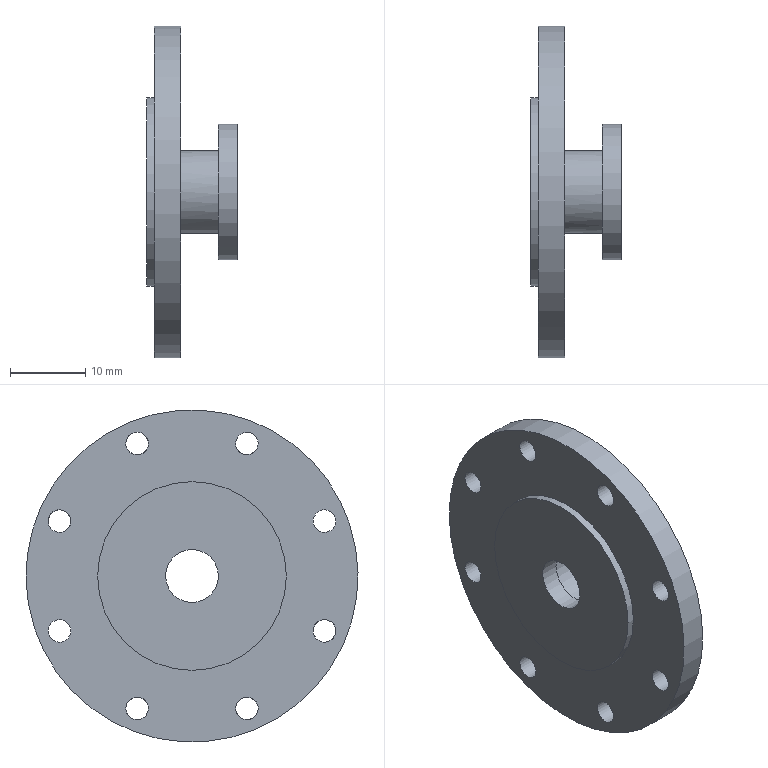Component | NX | END_CAP_3 | 1 solid | 26 faces | volume 5394 mm3 | cylinder 19 | plane 7 | commonest cylinder face diameters 3 x8 2.5 x4 11 x1 25 x1 44 x1 18 x1 8 x1 7 x1